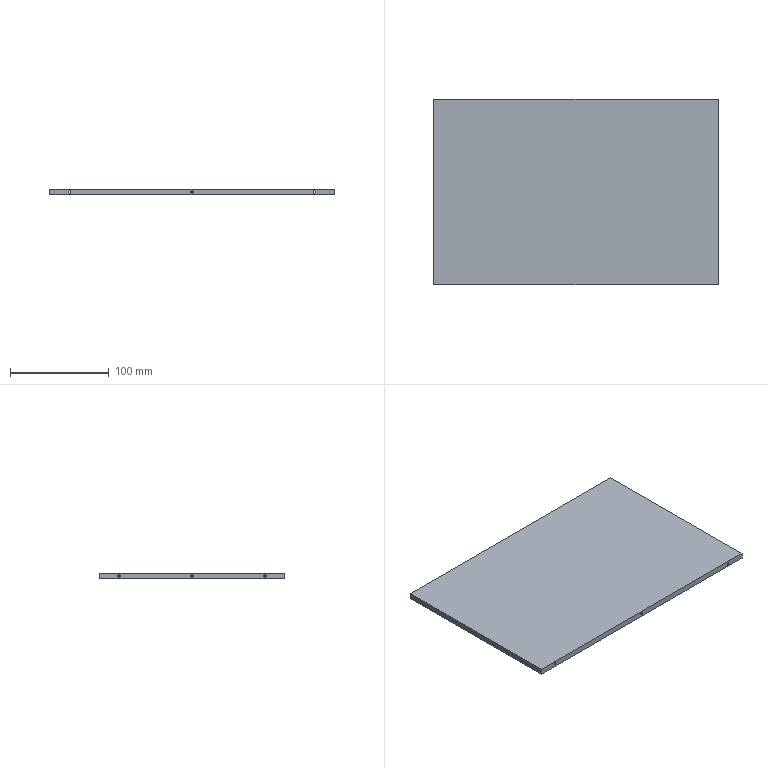CAM job | Mastercam | mm | 9 operations | part box 288 x 188 x 6
1. Contour (Ramp) | 12 - 12 平铣刀
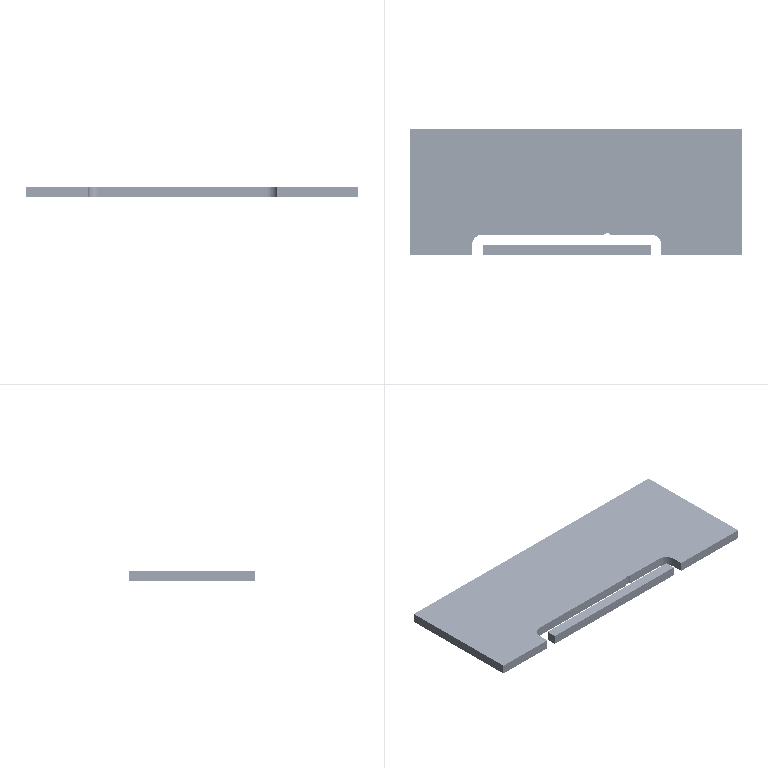2. Contour (2D) | 12 - 12 平铣刀
3. Contour (2D chamfer) | 7 - 4 倒角刀
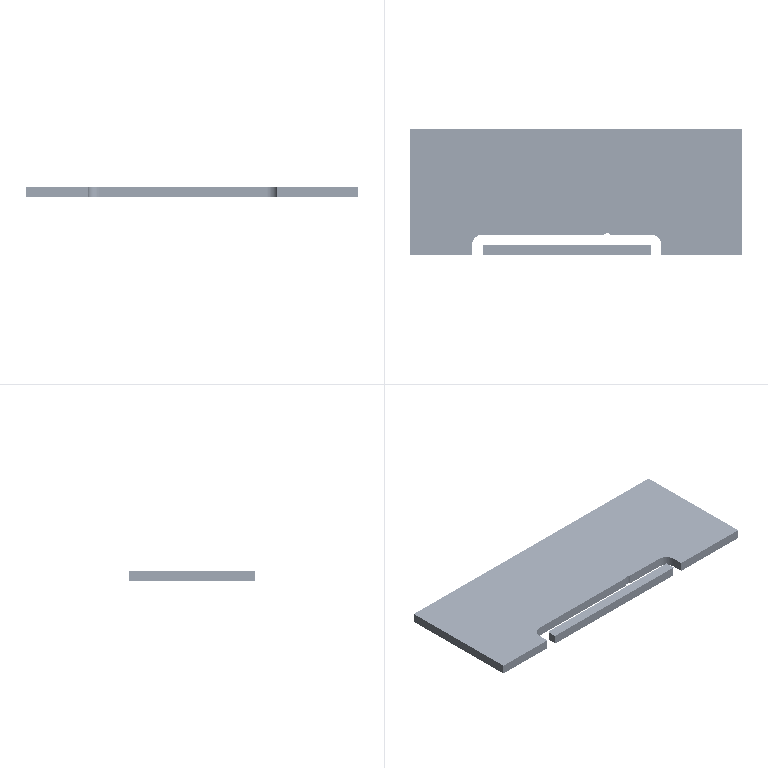4. Drill/Counterbore | 7 - 4 倒角刀
5. Peck Drill | 1 - 2.5 钻头
6. Contour (2D chamfer) | 7 - 4 倒角刀
7. Drill/Counterbore | 7 - 4 倒角刀
8. Peck Drill | 1 - 2.5 钻头
9. Contour (2D chamfer) | 7 - 4 倒角刀